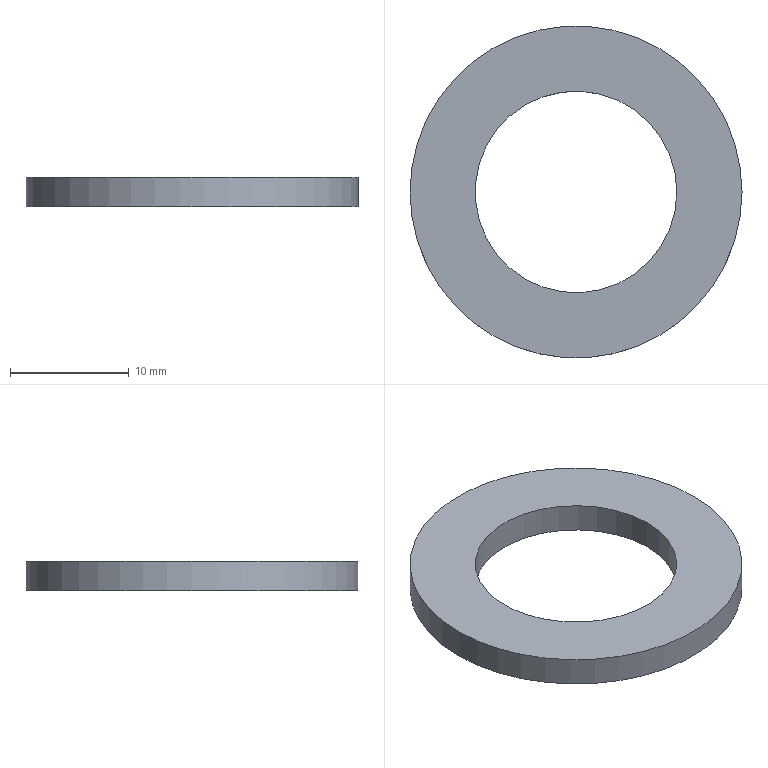Component | NX | GB-T848-2002_M16_2 | 1 solid | 4 faces | box 28 x 28 x 2.5 mm | volume 972 mm3 | cylinder 2 | plane 2 | commonest cylinder face diameters 28 x1 17 x1
STEP:
#1=CARTESIAN_POINT('',(0.,0.,0.));
#2=DIRECTION('',(0.,0.,1.));
#3=DIRECTION('',(1.,0.,0.));
#4=AXIS2_PLACEMENT_3D('',#1,#2,#3);
#5=CARTESIAN_POINT('',(125.,0.,217.5));
#6=VERTEX_POINT('',#5);
#7=CARTESIAN_POINT('',(111.,0.,217.5));
#8=DIRECTION('',(0.,0.,1.));
#9=DIRECTION('',(1.,0.,0.));
#10=AXIS2_PLACEMENT_3D('',#7,#8,#9);
#11=CIRCLE('',#10,14.);
#12=CARTESIAN_POINT('',(111.,0.,217.5));
#13=DIRECTION('',(0.,0.,-1.));
#14=DIRECTION('',(-1.,0.,0.));
#15=AXIS2_PLACEMENT_3D('',#12,#13,#14);
#16=CYLINDRICAL_SURFACE('',#15,14.);
#17=CARTESIAN_POINT('',(9.425,0.));
#18=DIRECTION('',(-1.,0.));
#19=VECTOR('',#18,1.);
#20=LINE('',#17,#19);
#21=(GEOMETRIC_REPRESENTATION_CONTEXT(2)PARAMETRIC_REPRESENTATION_CONTEXT()REPRESENTATION_CONTEXT('',''));
#22=DEFINITIONAL_REPRESENTATION('',(#20),#21);
#23=PCURVE('',#16,#22);
#24=CARTESIAN_POINT('',(111.,0.,217.5));
#25=DIRECTION('',(0.,0.,1.));
#26=DIRECTION('',(1.,0.,0.));
#27=AXIS2_PLACEMENT_3D('',#24,#25,#26);
#28=PLANE('',#27);
#29=CARTESIAN_POINT('',(0.,0.));
#30=DIRECTION('',(1.,0.));
#31=AXIS2_PLACEMENT_2D('',#29,#30);
#32=CIRCLE('',#31,14.);
#33=(GEOMETRIC_REPRESENTATION_CONTEXT(2)PARAMETRIC_REPRESENTATION_CONTEXT()REPRESENTATION_CONTEXT('',''));
#34=DEFINITIONAL_REPRESENTATION('',(#32),#33);
#35=PCURVE('',#28,#34);
#36=SURFACE_CURVE('',#11,(#23,#35),.PCURVE_S1.);
#37=EDGE_CURVE('',#6,#6,#36,.T.);
#38=ORIENTED_EDGE('',*,*,#37,.F.);
#39=CARTESIAN_POINT('',(125.,0.,215.));
#40=VERTEX_POINT('',#39);
#41=CARTESIAN_POINT('',(125.,0.,217.5));
#42=CARTESIAN_POINT('',(125.,0.,215.));
#43=B_SPLINE_CURVE_WITH_KNOTS('',1,(#41,#42),.UNSPECIFIED.,.F.,.F.,(2,2),(0.,2.5),.PIECEWISE_BEZIER_KNOTS.);
#44=CARTESIAN_POINT('',(9.425,0.));
#45=DIRECTION('',(0.,1.));
#46=VECTOR('',#45,1.);
#47=LINE('',#44,#46);
#48=(GEOMETRIC_REPRESENTATION_CONTEXT(2)PARAMETRIC_REPRESENTATION_CONTEXT()REPRESENTATION_CONTEXT('',''));
#49=DEFINITIONAL_REPRESENTATION('',(#47),#48);
#50=PCURVE('',#16,#49);
#51=CARTESIAN_POINT('',(3.142,0.));
#52=DIRECTION('',(0.,1.));
#53=VECTOR('',#52,1.);
#54=LINE('',#51,#53);
#55=(GEOMETRIC_REPRESENTATION_CONTEXT(2)PARAMETRIC_REPRESENTATION_CONTEXT()REPRESENTATION_CONTEXT('',''));
#56=DEFINITIONAL_REPRESENTATION('',(#54),#55);
#57=PCURVE('',#16,#56);
#58=SEAM_CURVE('',#43,(#50,#57),.PCURVE_S1.);
#59=EDGE_CURVE('',#6,#40,#58,.T.);
#60=ORIENTED_EDGE('',*,*,#59,.T.);
#61=CARTESIAN_POINT('',(111.,0.,215.));
#62=DIRECTION('',(0.,0.,1.));
#63=DIRECTION('',(1.,0.,0.));
#64=AXIS2_PLACEMENT_3D('',#61,#62,#63);
#65=CIRCLE('',#64,14.);
#66=CARTESIAN_POINT('',(9.425,2.5));
#67=DIRECTION('',(-1.,0.));
#68=VECTOR('',#67,1.);
#69=LINE('',#66,#68);
#70=(GEOMETRIC_REPRESENTATION_CONTEXT(2)PARAMETRIC_REPRESENTATION_CONTEXT()REPRESENTATION_CONTEXT('',''));
#71=DEFINITIONAL_REPRESENTATION('',(#69),#70);
#72=PCURVE('',#16,#71);
#73=CARTESIAN_POINT('',(111.,0.,215.));
#74=DIRECTION('',(0.,0.,1.));
#75=DIRECTION('',(1.,0.,0.));
#76=AXIS2_PLACEMENT_3D('',#73,#74,#75);
#77=PLANE('',#76);
#78=CARTESIAN_POINT('',(0.,0.));
#79=DIRECTION('',(1.,0.));
#80=AXIS2_PLACEMENT_2D('',#78,#79);
#81=CIRCLE('',#80,14.);
#82=(GEOMETRIC_REPRESENTATION_CONTEXT(2)PARAMETRIC_REPRESENTATION_CONTEXT()REPRESENTATION_CONTEXT('',''));
#83=DEFINITIONAL_REPRESENTATION('',(#81),#82);
#84=PCURVE('',#77,#83);
#85=SURFACE_CURVE('',#65,(#72,#84),.PCURVE_S1.);
#86=EDGE_CURVE('',#40,#40,#85,.T.);
#87=ORIENTED_EDGE('',*,*,#86,.T.);
#88=ORIENTED_EDGE('',*,*,#59,.F.);
#89=EDGE_LOOP('',(#38,#60,#87,#88));
#90=FACE_BOUND('',#89,.T.);
#91=ADVANCED_FACE('',(#90),#16,.T.);
#92=CARTESIAN_POINT('',(119.5,0.,217.5));
#93=VERTEX_POINT('',#92);
#94=CARTESIAN_POINT('',(111.,0.,217.5));
#95=DIRECTION('',(0.,0.,1.));
#96=DIRECTION('',(1.,0.,0.));
#97=AXIS2_PLACEMENT_3D('',#94,#95,#96);
#98=CIRCLE('',#97,8.5);
#99=CARTESIAN_POINT('',(111.,0.,217.5));
#100=DIRECTION('',(0.,0.,-1.));
#101=DIRECTION('',(-1.,0.,0.));
#102=AXIS2_PLACEMENT_3D('',#99,#100,#101);
#103=CYLINDRICAL_SURFACE('',#102,8.5);
#104=CARTESIAN_POINT('',(9.425,0.));
#105=DIRECTION('',(-1.,0.));
#106=VECTOR('',#105,1.);
#107=LINE('',#104,#106);
#108=(GEOMETRIC_REPRESENTATION_CONTEXT(2)PARAMETRIC_REPRESENTATION_CONTEXT()REPRESENTATION_CONTEXT('',''));
#109=DEFINITIONAL_REPRESENTATION('',(#107),#108);
#110=PCURVE('',#103,#109);
#111=CARTESIAN_POINT('',(0.,0.));
#112=DIRECTION('',(1.,0.));
#113=AXIS2_PLACEMENT_2D('',#111,#112);
#114=CIRCLE('',#113,8.5);
#115=(GEOMETRIC_REPRESENTATION_CONTEXT(2)PARAMETRIC_REPRESENTATION_CONTEXT()REPRESENTATION_CONTEXT('',''));
#116=DEFINITIONAL_REPRESENTATION('',(#114),#115);
#117=PCURVE('',#28,#116);
#118=SURFACE_CURVE('',#98,(#110,#117),.PCURVE_S1.);
#119=EDGE_CURVE('',#93,#93,#118,.T.);
#120=ORIENTED_EDGE('',*,*,#119,.F.);
#121=CARTESIAN_POINT('',(119.5,0.,215.));
#122=VERTEX_POINT('',#121);
#123=CARTESIAN_POINT('',(119.5,0.,217.5));
#124=CARTESIAN_POINT('',(119.5,0.,215.));
#125=B_SPLINE_CURVE_WITH_KNOTS('',1,(#123,#124),.UNSPECIFIED.,.F.,.F.,(2,2),(0.,2.5),.PIECEWISE_BEZIER_KNOTS.);
#126=CARTESIAN_POINT('',(9.425,0.));
#127=DIRECTION('',(0.,1.));
#128=VECTOR('',#127,1.);
#129=LINE('',#126,#128);
#130=(GEOMETRIC_REPRESENTATION_CONTEXT(2)PARAMETRIC_REPRESENTATION_CONTEXT()REPRESENTATION_CONTEXT('',''));
#131=DEFINITIONAL_REPRESENTATION('',(#129),#130);
#132=PCURVE('',#103,#131);
#133=CARTESIAN_POINT('',(3.142,0.));
#134=DIRECTION('',(0.,1.));
#135=VECTOR('',#134,1.);
#136=LINE('',#133,#135);
#137=(GEOMETRIC_REPRESENTATION_CONTEXT(2)PARAMETRIC_REPRESENTATION_CONTEXT()REPRESENTATION_CONTEXT('',''));
#138=DEFINITIONAL_REPRESENTATION('',(#136),#137);
#139=PCURVE('',#103,#138);
#140=SEAM_CURVE('',#125,(#132,#139),.PCURVE_S1.);
#141=EDGE_CURVE('',#93,#122,#140,.T.);
#142=ORIENTED_EDGE('',*,*,#141,.T.);
#143=CARTESIAN_POINT('',(111.,0.,215.));
#144=DIRECTION('',(0.,0.,1.));
#145=DIRECTION('',(1.,0.,0.));
#146=AXIS2_PLACEMENT_3D('',#143,#144,#145);
#147=CIRCLE('',#146,8.5);
#148=CARTESIAN_POINT('',(9.425,2.5));
#149=DIRECTION('',(-1.,0.));
#150=VECTOR('',#149,1.);
#151=LINE('',#148,#150);
#152=(GEOMETRIC_REPRESENTATION_CONTEXT(2)PARAMETRIC_REPRESENTATION_CONTEXT()REPRESENTATION_CONTEXT('',''));
#153=DEFINITIONAL_REPRESENTATION('',(#151),#152);
#154=PCURVE('',#103,#153);
#155=CARTESIAN_POINT('',(0.,0.));
#156=DIRECTION('',(1.,0.));
#157=AXIS2_PLACEMENT_2D('',#155,#156);
#158=CIRCLE('',#157,8.5);
#159=(GEOMETRIC_REPRESENTATION_CONTEXT(2)PARAMETRIC_REPRESENTATION_CONTEXT()REPRESENTATION_CONTEXT('',''));
#160=DEFINITIONAL_REPRESENTATION('',(#158),#159);
#161=PCURVE('',#77,#160);
#162=SURFACE_CURVE('',#147,(#154,#161),.PCURVE_S1.);
#163=EDGE_CURVE('',#122,#122,#162,.T.);
#164=ORIENTED_EDGE('',*,*,#163,.T.);
#165=ORIENTED_EDGE('',*,*,#141,.F.);
#166=EDGE_LOOP('',(#120,#142,#164,#165));
#167=FACE_BOUND('',#166,.F.);
#168=ADVANCED_FACE('',(#167),#103,.F.);
#169=ORIENTED_EDGE('',*,*,#37,.T.);
#170=EDGE_LOOP('',(#169));
#171=FACE_BOUND('',#170,.T.);
#172=ORIENTED_EDGE('',*,*,#119,.F.);
#173=EDGE_LOOP('',(#172));
#174=FACE_BOUND('',#173,.T.);
#175=ADVANCED_FACE('',(#171,#174),#28,.T.);
#176=ORIENTED_EDGE('',*,*,#86,.F.);
#177=EDGE_LOOP('',(#176));
#178=FACE_BOUND('',#177,.T.);
#179=ORIENTED_EDGE('',*,*,#163,.T.);
#180=EDGE_LOOP('',(#179));
#181=FACE_BOUND('',#180,.T.);
#182=ADVANCED_FACE('',(#178,#181),#77,.F.);
#183=CLOSED_SHELL('',(#91,#168,#175,#182));
#184=MANIFOLD_SOLID_BREP('',#183);
#185=(LENGTH_UNIT()NAMED_UNIT(*)SI_UNIT(.MILLI.,.METRE.));
#186=UNCERTAINTY_MEASURE_WITH_UNIT(LENGTH_MEASURE(0.00001),#185,'','');
#187=(NAMED_UNIT(*)PLANE_ANGLE_UNIT()SI_UNIT($,.RADIAN.));
#188=(NAMED_UNIT(*)SI_UNIT($,.STERADIAN.)SOLID_ANGLE_UNIT());
#189=(GEOMETRIC_REPRESENTATION_CONTEXT(3)GLOBAL_UNCERTAINTY_ASSIGNED_CONTEXT((#186))GLOBAL_UNIT_ASSIGNED_CONTEXT((#185,#187,#188))REPRESENTATION_CONTEXT('',''));
#190=ADVANCED_BREP_SHAPE_REPRESENTATION('',(#4,#184),#189);